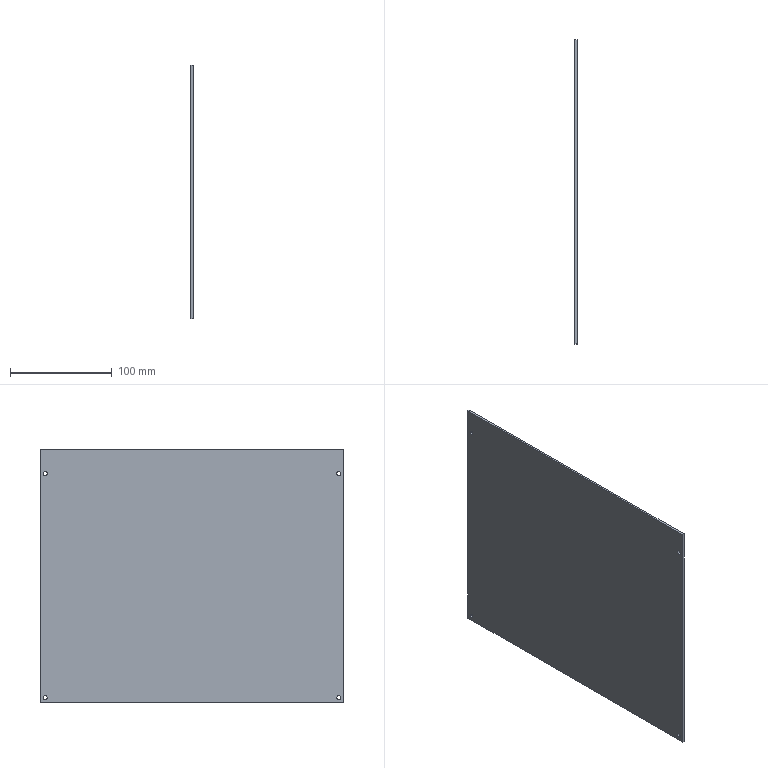Component | SolidWorks | LowerRightSurroundCoverPlate-1 | 1 solid | 14 faces | box 2 x 298 x 249 mm | volume 148303 mm3 | cylinder 8 | plane 6 | commonest cylinder face diameters 4 x8
build123d program:
from build123d import *

# Parameters (mm, degrees)
SKETCH1_W           = 249
SKETCH1_H           = 298
BOSS_EXTRUDE1_DEPTH = 2
SKETCH2_R           = 2
CUT_EXTRUDE1_DEPTH  = 2
LPATTERN1_COUNT     = 2
LPATTERN1_PITCH     = 220


with BuildPart() as part:
    # Sketch1 → Boss-Extrude1 (new body)
    with BuildSketch(Plane.XY):
        with Locations((-87.693, 114.719)):
            Rectangle(SKETCH1_W, SKETCH1_H)
    extrude(amount=BOSS_EXTRUDE1_DEPTH)

    # Sketch2 → Cut-Extrude1 (cut)
    with BuildSketch(Plane.XY.offset(2)):
        with Locations((31.807, 258.719)):
            Circle(SKETCH2_R)
        with Locations((31.807, -29.281)):
            Circle(SKETCH2_R)
    cut_extrude1 = extrude(amount=-CUT_EXTRUDE1_DEPTH, mode=Mode.SUBTRACT)

    # LPattern1: Cut-Extrude1 ×2
    with Locations(*[(-i * LPATTERN1_PITCH, 0, 0) for i in range(1, LPATTERN1_COUNT)]):
        add(cut_extrude1, mode=Mode.SUBTRACT)


solid = part.part

# Placed as in the assembly
solid = solid.moved(Location((783.45, -853.152, -210.712), (0, 90, 0)))
STEP:
#1=COLOUR_RGB('',0.7922,0.8196,0.9333);
#2=FILL_AREA_STYLE_COLOUR('',#1);
#3=FILL_AREA_STYLE('',(#2));
#4=SURFACE_STYLE_FILL_AREA(#3);
#5=SURFACE_SIDE_STYLE('',(#4));
#6=SURFACE_STYLE_USAGE(.BOTH.,#5);
#7=PRESENTATION_STYLE_ASSIGNMENT((#6));
#8=CARTESIAN_POINT('',(30.845,-34.741,-0.8078));
#9=VERTEX_POINT('',#8);
#10=CARTESIAN_POINT('',(30.845,-34.741,-0.9653));
#11=VERTEX_POINT('',#10);
#12=CARTESIAN_POINT('',(30.845,-34.741,-0.8866));
#13=DIRECTION('',(1.,0.,0.));
#14=DIRECTION('',(0.,0.,-1.));
#15=AXIS2_PLACEMENT_3D('',#12,#13,#14);
#16=CIRCLE('',#15,0.07874);
#17=EDGE_CURVE('',#9,#11,#16,.T.);
#18=ORIENTED_EDGE('',*,*,#17,.F.);
#19=CARTESIAN_POINT('',(30.923,-34.741,-0.8078));
#20=VERTEX_POINT('',#19);
#21=CARTESIAN_POINT('',(30.845,-34.741,-0.8078));
#22=DIRECTION('',(1.,0.,0.));
#23=VECTOR('',#22,39.37);
#24=LINE('',#21,#23);
#25=EDGE_CURVE('',#9,#20,#24,.T.);
#26=ORIENTED_EDGE('',*,*,#25,.T.);
#27=CARTESIAN_POINT('',(30.923,-34.741,-0.9653));
#28=VERTEX_POINT('',#27);
#29=CARTESIAN_POINT('',(30.923,-34.741,-0.8866));
#30=DIRECTION('',(1.,0.,0.));
#31=DIRECTION('',(0.,0.,-1.));
#32=AXIS2_PLACEMENT_3D('',#29,#30,#31);
#33=CIRCLE('',#32,0.07874);
#34=EDGE_CURVE('',#20,#28,#33,.T.);
#35=ORIENTED_EDGE('',*,*,#34,.T.);
#36=CARTESIAN_POINT('',(30.845,-34.741,-0.9653));
#37=DIRECTION('',(1.,0.,0.));
#38=VECTOR('',#37,39.37);
#39=LINE('',#36,#38);
#40=EDGE_CURVE('',#11,#28,#39,.T.);
#41=ORIENTED_EDGE('',*,*,#40,.F.);
#42=EDGE_LOOP('',(#18,#26,#35,#41));
#43=FACE_OUTER_BOUND('',#42,.T.);
#44=CARTESIAN_POINT('',(30.845,-34.741,-0.8866));
#45=DIRECTION('',(1.,0.,0.));
#46=DIRECTION('',(0.,0.,-1.));
#47=AXIS2_PLACEMENT_3D('',#44,#45,#46);
#48=CYLINDRICAL_SURFACE('',#47,0.07874);
#49=ADVANCED_FACE('',(#43),#48,.F.);
#50=CARTESIAN_POINT('',(30.845,-23.403,-0.8078));
#51=VERTEX_POINT('',#50);
#52=CARTESIAN_POINT('',(30.845,-23.403,-0.9653));
#53=VERTEX_POINT('',#52);
#54=CARTESIAN_POINT('',(30.845,-23.403,-0.8866));
#55=DIRECTION('',(1.,0.,0.));
#56=DIRECTION('',(0.,0.,-1.));
#57=AXIS2_PLACEMENT_3D('',#54,#55,#56);
#58=CIRCLE('',#57,0.07874);
#59=EDGE_CURVE('',#51,#53,#58,.T.);
#60=ORIENTED_EDGE('',*,*,#59,.F.);
#61=CARTESIAN_POINT('',(30.923,-23.403,-0.8078));
#62=VERTEX_POINT('',#61);
#63=CARTESIAN_POINT('',(30.845,-23.403,-0.8078));
#64=DIRECTION('',(1.,0.,0.));
#65=VECTOR('',#64,39.37);
#66=LINE('',#63,#65);
#67=EDGE_CURVE('',#51,#62,#66,.T.);
#68=ORIENTED_EDGE('',*,*,#67,.T.);
#69=CARTESIAN_POINT('',(30.923,-23.403,-0.9653));
#70=VERTEX_POINT('',#69);
#71=CARTESIAN_POINT('',(30.923,-23.403,-0.8866));
#72=DIRECTION('',(1.,0.,0.));
#73=DIRECTION('',(0.,0.,-1.));
#74=AXIS2_PLACEMENT_3D('',#71,#72,#73);
#75=CIRCLE('',#74,0.07874);
#76=EDGE_CURVE('',#62,#70,#75,.T.);
#77=ORIENTED_EDGE('',*,*,#76,.T.);
#78=CARTESIAN_POINT('',(30.845,-23.403,-0.9653));
#79=DIRECTION('',(1.,0.,0.));
#80=VECTOR('',#79,39.37);
#81=LINE('',#78,#80);
#82=EDGE_CURVE('',#53,#70,#81,.T.);
#83=ORIENTED_EDGE('',*,*,#82,.F.);
#84=EDGE_LOOP('',(#60,#68,#77,#83));
#85=FACE_OUTER_BOUND('',#84,.T.);
#86=CARTESIAN_POINT('',(30.845,-23.403,-0.8866));
#87=DIRECTION('',(1.,0.,0.));
#88=DIRECTION('',(0.,0.,-1.));
#89=AXIS2_PLACEMENT_3D('',#86,#87,#88);
#90=CYLINDRICAL_SURFACE('',#89,0.07874);
#91=ADVANCED_FACE('',(#85),#90,.F.);
#92=CARTESIAN_POINT('',(30.845,-34.741,-9.469));
#93=VERTEX_POINT('',#92);
#94=CARTESIAN_POINT('',(30.845,-34.741,-9.627));
#95=VERTEX_POINT('',#94);
#96=CARTESIAN_POINT('',(30.845,-34.741,-9.548));
#97=DIRECTION('',(1.,0.,0.));
#98=DIRECTION('',(0.,0.,-1.));
#99=AXIS2_PLACEMENT_3D('',#96,#97,#98);
#100=CIRCLE('',#99,0.07874);
#101=EDGE_CURVE('',#93,#95,#100,.T.);
#102=ORIENTED_EDGE('',*,*,#101,.F.);
#103=CARTESIAN_POINT('',(30.923,-34.741,-9.469));
#104=VERTEX_POINT('',#103);
#105=CARTESIAN_POINT('',(30.845,-34.741,-9.469));
#106=DIRECTION('',(1.,0.,0.));
#107=VECTOR('',#106,39.37);
#108=LINE('',#105,#107);
#109=EDGE_CURVE('',#93,#104,#108,.T.);
#110=ORIENTED_EDGE('',*,*,#109,.T.);
#111=CARTESIAN_POINT('',(30.923,-34.741,-9.627));
#112=VERTEX_POINT('',#111);
#113=CARTESIAN_POINT('',(30.923,-34.741,-9.548));
#114=DIRECTION('',(1.,0.,0.));
#115=DIRECTION('',(0.,0.,-1.));
#116=AXIS2_PLACEMENT_3D('',#113,#114,#115);
#117=CIRCLE('',#116,0.07874);
#118=EDGE_CURVE('',#104,#112,#117,.T.);
#119=ORIENTED_EDGE('',*,*,#118,.T.);
#120=CARTESIAN_POINT('',(30.845,-34.741,-9.627));
#121=DIRECTION('',(1.,0.,0.));
#122=VECTOR('',#121,39.37);
#123=LINE('',#120,#122);
#124=EDGE_CURVE('',#95,#112,#123,.T.);
#125=ORIENTED_EDGE('',*,*,#124,.F.);
#126=EDGE_LOOP('',(#102,#110,#119,#125));
#127=FACE_OUTER_BOUND('',#126,.T.);
#128=CARTESIAN_POINT('',(30.845,-34.741,-9.548));
#129=DIRECTION('',(1.,0.,0.));
#130=DIRECTION('',(0.,0.,-1.));
#131=AXIS2_PLACEMENT_3D('',#128,#129,#130);
#132=CYLINDRICAL_SURFACE('',#131,0.07874);
#133=ADVANCED_FACE('',(#127),#132,.F.);
#134=CARTESIAN_POINT('',(30.845,-23.403,-9.469));
#135=VERTEX_POINT('',#134);
#136=CARTESIAN_POINT('',(30.845,-23.403,-9.627));
#137=VERTEX_POINT('',#136);
#138=CARTESIAN_POINT('',(30.845,-23.403,-9.548));
#139=DIRECTION('',(1.,0.,0.));
#140=DIRECTION('',(0.,0.,-1.));
#141=AXIS2_PLACEMENT_3D('',#138,#139,#140);
#142=CIRCLE('',#141,0.07874);
#143=EDGE_CURVE('',#135,#137,#142,.T.);
#144=ORIENTED_EDGE('',*,*,#143,.F.);
#145=CARTESIAN_POINT('',(30.923,-23.403,-9.469));
#146=VERTEX_POINT('',#145);
#147=CARTESIAN_POINT('',(30.845,-23.403,-9.469));
#148=DIRECTION('',(1.,0.,0.));
#149=VECTOR('',#148,39.37);
#150=LINE('',#147,#149);
#151=EDGE_CURVE('',#135,#146,#150,.T.);
#152=ORIENTED_EDGE('',*,*,#151,.T.);
#153=CARTESIAN_POINT('',(30.923,-23.403,-9.627));
#154=VERTEX_POINT('',#153);
#155=CARTESIAN_POINT('',(30.923,-23.403,-9.548));
#156=DIRECTION('',(1.,0.,0.));
#157=DIRECTION('',(0.,0.,-1.));
#158=AXIS2_PLACEMENT_3D('',#155,#156,#157);
#159=CIRCLE('',#158,0.07874);
#160=EDGE_CURVE('',#146,#154,#159,.T.);
#161=ORIENTED_EDGE('',*,*,#160,.T.);
#162=CARTESIAN_POINT('',(30.845,-23.403,-9.627));
#163=DIRECTION('',(1.,0.,0.));
#164=VECTOR('',#163,39.37);
#165=LINE('',#162,#164);
#166=EDGE_CURVE('',#137,#154,#165,.T.);
#167=ORIENTED_EDGE('',*,*,#166,.F.);
#168=EDGE_LOOP('',(#144,#152,#161,#167));
#169=FACE_OUTER_BOUND('',#168,.T.);
#170=CARTESIAN_POINT('',(30.845,-23.403,-9.548));
#171=DIRECTION('',(1.,0.,0.));
#172=DIRECTION('',(0.,0.,-1.));
#173=AXIS2_PLACEMENT_3D('',#170,#171,#172);
#174=CYLINDRICAL_SURFACE('',#173,0.07874);
#175=ADVANCED_FACE('',(#169),#174,.F.);
#176=CARTESIAN_POINT('',(30.845,-34.938,-9.745));
#177=VERTEX_POINT('',#176);
#178=CARTESIAN_POINT('',(30.845,-23.206,-9.745));
#179=VERTEX_POINT('',#178);
#180=CARTESIAN_POINT('',(30.845,-23.206,-9.745));
#181=DIRECTION('',(-0.,1.,0.));
#182=VECTOR('',#181,39.37);
#183=LINE('',#180,#182);
#184=EDGE_CURVE('',#177,#179,#183,.T.);
#185=ORIENTED_EDGE('',*,*,#184,.T.);
#186=CARTESIAN_POINT('',(30.923,-23.206,-9.745));
#187=VERTEX_POINT('',#186);
#188=CARTESIAN_POINT('',(30.923,-23.206,-9.745));
#189=DIRECTION('',(-1.,-0.,-0.));
#190=VECTOR('',#189,39.37);
#191=LINE('',#188,#190);
#192=EDGE_CURVE('',#187,#179,#191,.T.);
#193=ORIENTED_EDGE('',*,*,#192,.F.);
#194=CARTESIAN_POINT('',(30.923,-34.938,-9.745));
#195=VERTEX_POINT('',#194);
#196=CARTESIAN_POINT('',(30.923,-23.206,-9.745));
#197=DIRECTION('',(-0.,1.,0.));
#198=VECTOR('',#197,39.37);
#199=LINE('',#196,#198);
#200=EDGE_CURVE('',#195,#187,#199,.T.);
#201=ORIENTED_EDGE('',*,*,#200,.F.);
#202=CARTESIAN_POINT('',(30.923,-34.938,-9.745));
#203=DIRECTION('',(-1.,-0.,-0.));
#204=VECTOR('',#203,39.37);
#205=LINE('',#202,#204);
#206=EDGE_CURVE('',#195,#177,#205,.T.);
#207=ORIENTED_EDGE('',*,*,#206,.T.);
#208=EDGE_LOOP('',(#185,#193,#201,#207));
#209=FACE_OUTER_BOUND('',#208,.T.);
#210=CARTESIAN_POINT('',(30.923,-23.206,-9.745));
#211=DIRECTION('',(-0.,-0.,1.));
#212=DIRECTION('',(0.,-1.,-0.));
#213=AXIS2_PLACEMENT_3D('',#210,#211,#212);
#214=PLANE('',#213);
#215=ADVANCED_FACE('',(#209),#214,.F.);
#216=CARTESIAN_POINT('',(30.845,-23.206,0.0583));
#217=VERTEX_POINT('',#216);
#218=CARTESIAN_POINT('',(30.845,-23.206,0.0583));
#219=DIRECTION('',(-0.,0.,1.));
#220=VECTOR('',#219,39.37);
#221=LINE('',#218,#220);
#222=EDGE_CURVE('',#179,#217,#221,.T.);
#223=ORIENTED_EDGE('',*,*,#222,.T.);
#224=CARTESIAN_POINT('',(30.923,-23.206,0.0583));
#225=VERTEX_POINT('',#224);
#226=CARTESIAN_POINT('',(30.923,-23.206,0.0583));
#227=DIRECTION('',(-1.,-0.,-0.));
#228=VECTOR('',#227,39.37);
#229=LINE('',#226,#228);
#230=EDGE_CURVE('',#225,#217,#229,.T.);
#231=ORIENTED_EDGE('',*,*,#230,.F.);
#232=CARTESIAN_POINT('',(30.923,-23.206,0.0583));
#233=DIRECTION('',(-0.,0.,1.));
#234=VECTOR('',#233,39.37);
#235=LINE('',#232,#234);
#236=EDGE_CURVE('',#187,#225,#235,.T.);
#237=ORIENTED_EDGE('',*,*,#236,.F.);
#238=ORIENTED_EDGE('',*,*,#192,.T.);
#239=EDGE_LOOP('',(#223,#231,#237,#238));
#240=FACE_OUTER_BOUND('',#239,.T.);
#241=CARTESIAN_POINT('',(30.923,-23.206,0.0583));
#242=DIRECTION('',(0.,-1.,0.));
#243=DIRECTION('',(-1.,-0.,-0.));
#244=AXIS2_PLACEMENT_3D('',#241,#242,#243);
#245=PLANE('',#244);
#246=ADVANCED_FACE('',(#240),#245,.F.);
#247=CARTESIAN_POINT('',(30.845,-34.938,0.0583));
#248=VERTEX_POINT('',#247);
#249=CARTESIAN_POINT('',(30.845,-23.206,0.0583));
#250=DIRECTION('',(0.,-1.,0.));
#251=VECTOR('',#250,39.37);
#252=LINE('',#249,#251);
#253=EDGE_CURVE('',#217,#248,#252,.T.);
#254=ORIENTED_EDGE('',*,*,#253,.T.);
#255=CARTESIAN_POINT('',(30.923,-34.938,0.0583));
#256=VERTEX_POINT('',#255);
#257=CARTESIAN_POINT('',(30.923,-34.938,0.0583));
#258=DIRECTION('',(-1.,-0.,-0.));
#259=VECTOR('',#258,39.37);
#260=LINE('',#257,#259);
#261=EDGE_CURVE('',#256,#248,#260,.T.);
#262=ORIENTED_EDGE('',*,*,#261,.F.);
#263=CARTESIAN_POINT('',(30.923,-23.206,0.0583));
#264=DIRECTION('',(0.,-1.,0.));
#265=VECTOR('',#264,39.37);
#266=LINE('',#263,#265);
#267=EDGE_CURVE('',#225,#256,#266,.T.);
#268=ORIENTED_EDGE('',*,*,#267,.F.);
#269=ORIENTED_EDGE('',*,*,#230,.T.);
#270=EDGE_LOOP('',(#254,#262,#268,#269));
#271=FACE_OUTER_BOUND('',#270,.T.);
#272=CARTESIAN_POINT('',(30.923,-23.206,0.0583));
#273=DIRECTION('',(0.,-0.,-1.));
#274=DIRECTION('',(-0.,1.,-0.));
#275=AXIS2_PLACEMENT_3D('',#272,#273,#274);
#276=PLANE('',#275);
#277=ADVANCED_FACE('',(#271),#276,.F.);
#278=CARTESIAN_POINT('',(30.845,-34.938,0.0583));
#279=DIRECTION('',(0.,-0.,-1.));
#280=VECTOR('',#279,39.37);
#281=LINE('',#278,#280);
#282=EDGE_CURVE('',#248,#177,#281,.T.);
#283=ORIENTED_EDGE('',*,*,#282,.T.);
#284=ORIENTED_EDGE('',*,*,#206,.F.);
#285=CARTESIAN_POINT('',(30.923,-34.938,0.0583));
#286=DIRECTION('',(0.,-0.,-1.));
#287=VECTOR('',#286,39.37);
#288=LINE('',#285,#287);
#289=EDGE_CURVE('',#256,#195,#288,.T.);
#290=ORIENTED_EDGE('',*,*,#289,.F.);
#291=ORIENTED_EDGE('',*,*,#261,.T.);
#292=EDGE_LOOP('',(#283,#284,#290,#291));
#293=FACE_OUTER_BOUND('',#292,.T.);
#294=CARTESIAN_POINT('',(30.923,-34.938,0.0583));
#295=DIRECTION('',(-0.,1.,-0.));
#296=DIRECTION('',(1.,0.,0.));
#297=AXIS2_PLACEMENT_3D('',#294,#295,#296);
#298=PLANE('',#297);
#299=ADVANCED_FACE('',(#293),#298,.F.);
#300=CARTESIAN_POINT('',(30.923,-34.741,-0.8866));
#301=DIRECTION('',(1.,0.,0.));
#302=DIRECTION('',(0.,0.,-1.));
#303=AXIS2_PLACEMENT_3D('',#300,#301,#302);
#304=CIRCLE('',#303,0.07874);
#305=EDGE_CURVE('',#28,#20,#304,.T.);
#306=ORIENTED_EDGE('',*,*,#305,.F.);
#307=ORIENTED_EDGE('',*,*,#34,.F.);
#308=EDGE_LOOP('',(#306,#307));
#309=FACE_BOUND('',#308,.T.);
#310=CARTESIAN_POINT('',(30.923,-23.403,-0.8866));
#311=DIRECTION('',(1.,0.,0.));
#312=DIRECTION('',(0.,0.,-1.));
#313=AXIS2_PLACEMENT_3D('',#310,#311,#312);
#314=CIRCLE('',#313,0.07874);
#315=EDGE_CURVE('',#70,#62,#314,.T.);
#316=ORIENTED_EDGE('',*,*,#315,.F.);
#317=ORIENTED_EDGE('',*,*,#76,.F.);
#318=EDGE_LOOP('',(#316,#317));
#319=FACE_BOUND('',#318,.T.);
#320=CARTESIAN_POINT('',(30.923,-34.741,-9.548));
#321=DIRECTION('',(1.,0.,0.));
#322=DIRECTION('',(0.,0.,-1.));
#323=AXIS2_PLACEMENT_3D('',#320,#321,#322);
#324=CIRCLE('',#323,0.07874);
#325=EDGE_CURVE('',#112,#104,#324,.T.);
#326=ORIENTED_EDGE('',*,*,#325,.F.);
#327=ORIENTED_EDGE('',*,*,#118,.F.);
#328=EDGE_LOOP('',(#326,#327));
#329=FACE_BOUND('',#328,.T.);
#330=CARTESIAN_POINT('',(30.923,-23.403,-9.548));
#331=DIRECTION('',(1.,0.,0.));
#332=DIRECTION('',(0.,0.,-1.));
#333=AXIS2_PLACEMENT_3D('',#330,#331,#332);
#334=CIRCLE('',#333,0.07874);
#335=EDGE_CURVE('',#154,#146,#334,.T.);
#336=ORIENTED_EDGE('',*,*,#335,.F.);
#337=ORIENTED_EDGE('',*,*,#160,.F.);
#338=EDGE_LOOP('',(#336,#337));
#339=FACE_BOUND('',#338,.T.);
#340=ORIENTED_EDGE('',*,*,#200,.T.);
#341=ORIENTED_EDGE('',*,*,#236,.T.);
#342=ORIENTED_EDGE('',*,*,#267,.T.);
#343=ORIENTED_EDGE('',*,*,#289,.T.);
#344=EDGE_LOOP('',(#340,#341,#342,#343));
#345=FACE_OUTER_BOUND('',#344,.T.);
#346=CARTESIAN_POINT('',(30.923,-33.589,-8.296));
#347=DIRECTION('',(1.,0.,0.));
#348=DIRECTION('',(0.,-0.,-1.));
#349=AXIS2_PLACEMENT_3D('',#346,#347,#348);
#350=PLANE('',#349);
#351=ADVANCED_FACE('',(#309,#319,#329,#339,#345),#350,.T.);
#352=CARTESIAN_POINT('',(30.845,-34.741,-0.8866));
#353=DIRECTION('',(1.,0.,0.));
#354=DIRECTION('',(0.,0.,-1.));
#355=AXIS2_PLACEMENT_3D('',#352,#353,#354);
#356=CIRCLE('',#355,0.07874);
#357=EDGE_CURVE('',#11,#9,#356,.T.);
#358=ORIENTED_EDGE('',*,*,#357,.T.);
#359=ORIENTED_EDGE('',*,*,#17,.T.);
#360=EDGE_LOOP('',(#358,#359));
#361=FACE_BOUND('',#360,.T.);
#362=CARTESIAN_POINT('',(30.845,-23.403,-0.8866));
#363=DIRECTION('',(1.,0.,0.));
#364=DIRECTION('',(0.,0.,-1.));
#365=AXIS2_PLACEMENT_3D('',#362,#363,#364);
#366=CIRCLE('',#365,0.07874);
#367=EDGE_CURVE('',#53,#51,#366,.T.);
#368=ORIENTED_EDGE('',*,*,#367,.T.);
#369=ORIENTED_EDGE('',*,*,#59,.T.);
#370=EDGE_LOOP('',(#368,#369));
#371=FACE_BOUND('',#370,.T.);
#372=CARTESIAN_POINT('',(30.845,-34.741,-9.548));
#373=DIRECTION('',(1.,0.,0.));
#374=DIRECTION('',(0.,0.,-1.));
#375=AXIS2_PLACEMENT_3D('',#372,#373,#374);
#376=CIRCLE('',#375,0.07874);
#377=EDGE_CURVE('',#95,#93,#376,.T.);
#378=ORIENTED_EDGE('',*,*,#377,.T.);
#379=ORIENTED_EDGE('',*,*,#101,.T.);
#380=EDGE_LOOP('',(#378,#379));
#381=FACE_BOUND('',#380,.T.);
#382=CARTESIAN_POINT('',(30.845,-23.403,-9.548));
#383=DIRECTION('',(1.,0.,0.));
#384=DIRECTION('',(0.,0.,-1.));
#385=AXIS2_PLACEMENT_3D('',#382,#383,#384);
#386=CIRCLE('',#385,0.07874);
#387=EDGE_CURVE('',#137,#135,#386,.T.);
#388=ORIENTED_EDGE('',*,*,#387,.T.);
#389=ORIENTED_EDGE('',*,*,#143,.T.);
#390=EDGE_LOOP('',(#388,#389));
#391=FACE_BOUND('',#390,.T.);
#392=ORIENTED_EDGE('',*,*,#184,.F.);
#393=ORIENTED_EDGE('',*,*,#282,.F.);
#394=ORIENTED_EDGE('',*,*,#253,.F.);
#395=ORIENTED_EDGE('',*,*,#222,.F.);
#396=EDGE_LOOP('',(#392,#393,#394,#395));
#397=FACE_OUTER_BOUND('',#396,.T.);
#398=CARTESIAN_POINT('',(30.845,-33.589,-8.296));
#399=DIRECTION('',(1.,0.,0.));
#400=DIRECTION('',(0.,-0.,-1.));
#401=AXIS2_PLACEMENT_3D('',#398,#399,#400);
#402=PLANE('',#401);
#403=ADVANCED_FACE('',(#361,#371,#381,#391,#397),#402,.F.);
#404=ORIENTED_EDGE('',*,*,#151,.F.);
#405=ORIENTED_EDGE('',*,*,#387,.F.);
#406=ORIENTED_EDGE('',*,*,#166,.T.);
#407=ORIENTED_EDGE('',*,*,#335,.T.);
#408=EDGE_LOOP('',(#404,#405,#406,#407));
#409=FACE_OUTER_BOUND('',#408,.T.);
#410=CARTESIAN_POINT('',(30.845,-23.403,-9.548));
#411=DIRECTION('',(1.,0.,0.));
#412=DIRECTION('',(0.,0.,-1.));
#413=AXIS2_PLACEMENT_3D('',#410,#411,#412);
#414=CYLINDRICAL_SURFACE('',#413,0.07874);
#415=ADVANCED_FACE('',(#409),#414,.F.);
#416=ORIENTED_EDGE('',*,*,#109,.F.);
#417=ORIENTED_EDGE('',*,*,#377,.F.);
#418=ORIENTED_EDGE('',*,*,#124,.T.);
#419=ORIENTED_EDGE('',*,*,#325,.T.);
#420=EDGE_LOOP('',(#416,#417,#418,#419));
#421=FACE_OUTER_BOUND('',#420,.T.);
#422=CARTESIAN_POINT('',(30.845,-34.741,-9.548));
#423=DIRECTION('',(1.,0.,0.));
#424=DIRECTION('',(0.,0.,-1.));
#425=AXIS2_PLACEMENT_3D('',#422,#423,#424);
#426=CYLINDRICAL_SURFACE('',#425,0.07874);
#427=ADVANCED_FACE('',(#421),#426,.F.);
#428=ORIENTED_EDGE('',*,*,#67,.F.);
#429=ORIENTED_EDGE('',*,*,#367,.F.);
#430=ORIENTED_EDGE('',*,*,#82,.T.);
#431=ORIENTED_EDGE('',*,*,#315,.T.);
#432=EDGE_LOOP('',(#428,#429,#430,#431));
#433=FACE_OUTER_BOUND('',#432,.T.);
#434=CARTESIAN_POINT('',(30.845,-23.403,-0.8866));
#435=DIRECTION('',(1.,0.,0.));
#436=DIRECTION('',(0.,0.,-1.));
#437=AXIS2_PLACEMENT_3D('',#434,#435,#436);
#438=CYLINDRICAL_SURFACE('',#437,0.07874);
#439=ADVANCED_FACE('',(#433),#438,.F.);
#440=ORIENTED_EDGE('',*,*,#25,.F.);
#441=ORIENTED_EDGE('',*,*,#357,.F.);
#442=ORIENTED_EDGE('',*,*,#40,.T.);
#443=ORIENTED_EDGE('',*,*,#305,.T.);
#444=EDGE_LOOP('',(#440,#441,#442,#443));
#445=FACE_OUTER_BOUND('',#444,.T.);
#446=CARTESIAN_POINT('',(30.845,-34.741,-0.8866));
#447=DIRECTION('',(1.,0.,0.));
#448=DIRECTION('',(0.,0.,-1.));
#449=AXIS2_PLACEMENT_3D('',#446,#447,#448);
#450=CYLINDRICAL_SURFACE('',#449,0.07874);
#451=ADVANCED_FACE('',(#445),#450,.F.);
#452=CLOSED_SHELL('',(#49,#91,#133,#175,#215,#246,#277,#299,#351,#403,#415,#427,#439,#451));
#453=MANIFOLD_SOLID_BREP('',#452);
#454=STYLED_ITEM('',(#7),#453);
#455=PRESENTATION_LAYER_ASSIGNMENT('','',(#454));
#456=CARTESIAN_POINT('',(0.,0.,0.));
#457=DIRECTION('',(0.,0.,1.));
#458=DIRECTION('',(1.,0.,0.));
#459=AXIS2_PLACEMENT_3D('',#456,#457,#458);
#460=(LENGTH_UNIT()NAMED_UNIT(*)SI_UNIT($,.METRE.));
#461=LENGTH_MEASURE_WITH_UNIT(LENGTH_MEASURE(0.0254),#460);
#462=DIMENSIONAL_EXPONENTS(1.,0.,0.,0.,0.,0.,0.);
#463=(CONVERSION_BASED_UNIT('',#461)LENGTH_UNIT()NAMED_UNIT(#462));
#464=UNCERTAINTY_MEASURE_WITH_UNIT(LENGTH_MEASURE(0.00001),#463,'','');
#465=(NAMED_UNIT(*)PLANE_ANGLE_UNIT()SI_UNIT($,.RADIAN.));
#466=(NAMED_UNIT(*)SI_UNIT($,.STERADIAN.)SOLID_ANGLE_UNIT());
#467=(GEOMETRIC_REPRESENTATION_CONTEXT(3)GLOBAL_UNCERTAINTY_ASSIGNED_CONTEXT((#464))GLOBAL_UNIT_ASSIGNED_CONTEXT((#463,#465,#466))REPRESENTATION_CONTEXT('',''));
#468=ADVANCED_BREP_SHAPE_REPRESENTATION('',(#453,#459),#467);
#469=(LENGTH_UNIT()NAMED_UNIT(*)SI_UNIT($,.METRE.));
#470=LENGTH_MEASURE_WITH_UNIT(LENGTH_MEASURE(0.0254),#469);
#471=DIMENSIONAL_EXPONENTS(1.,0.,0.,0.,0.,0.,0.);
#472=(CONVERSION_BASED_UNIT('',#470)LENGTH_UNIT()NAMED_UNIT(#471));
#473=UNCERTAINTY_MEASURE_WITH_UNIT(LENGTH_MEASURE(0.00001),#472,'','');
#474=(NAMED_UNIT(*)PLANE_ANGLE_UNIT()SI_UNIT($,.RADIAN.));
#475=(NAMED_UNIT(*)SI_UNIT($,.STERADIAN.)SOLID_ANGLE_UNIT());
#476=(GEOMETRIC_REPRESENTATION_CONTEXT(3)GLOBAL_UNCERTAINTY_ASSIGNED_CONTEXT((#473))GLOBAL_UNIT_ASSIGNED_CONTEXT((#472,#474,#475))REPRESENTATION_CONTEXT('',''));
#477=MECHANICAL_DESIGN_GEOMETRIC_PRESENTATION_REPRESENTATION('',(#454),#476);